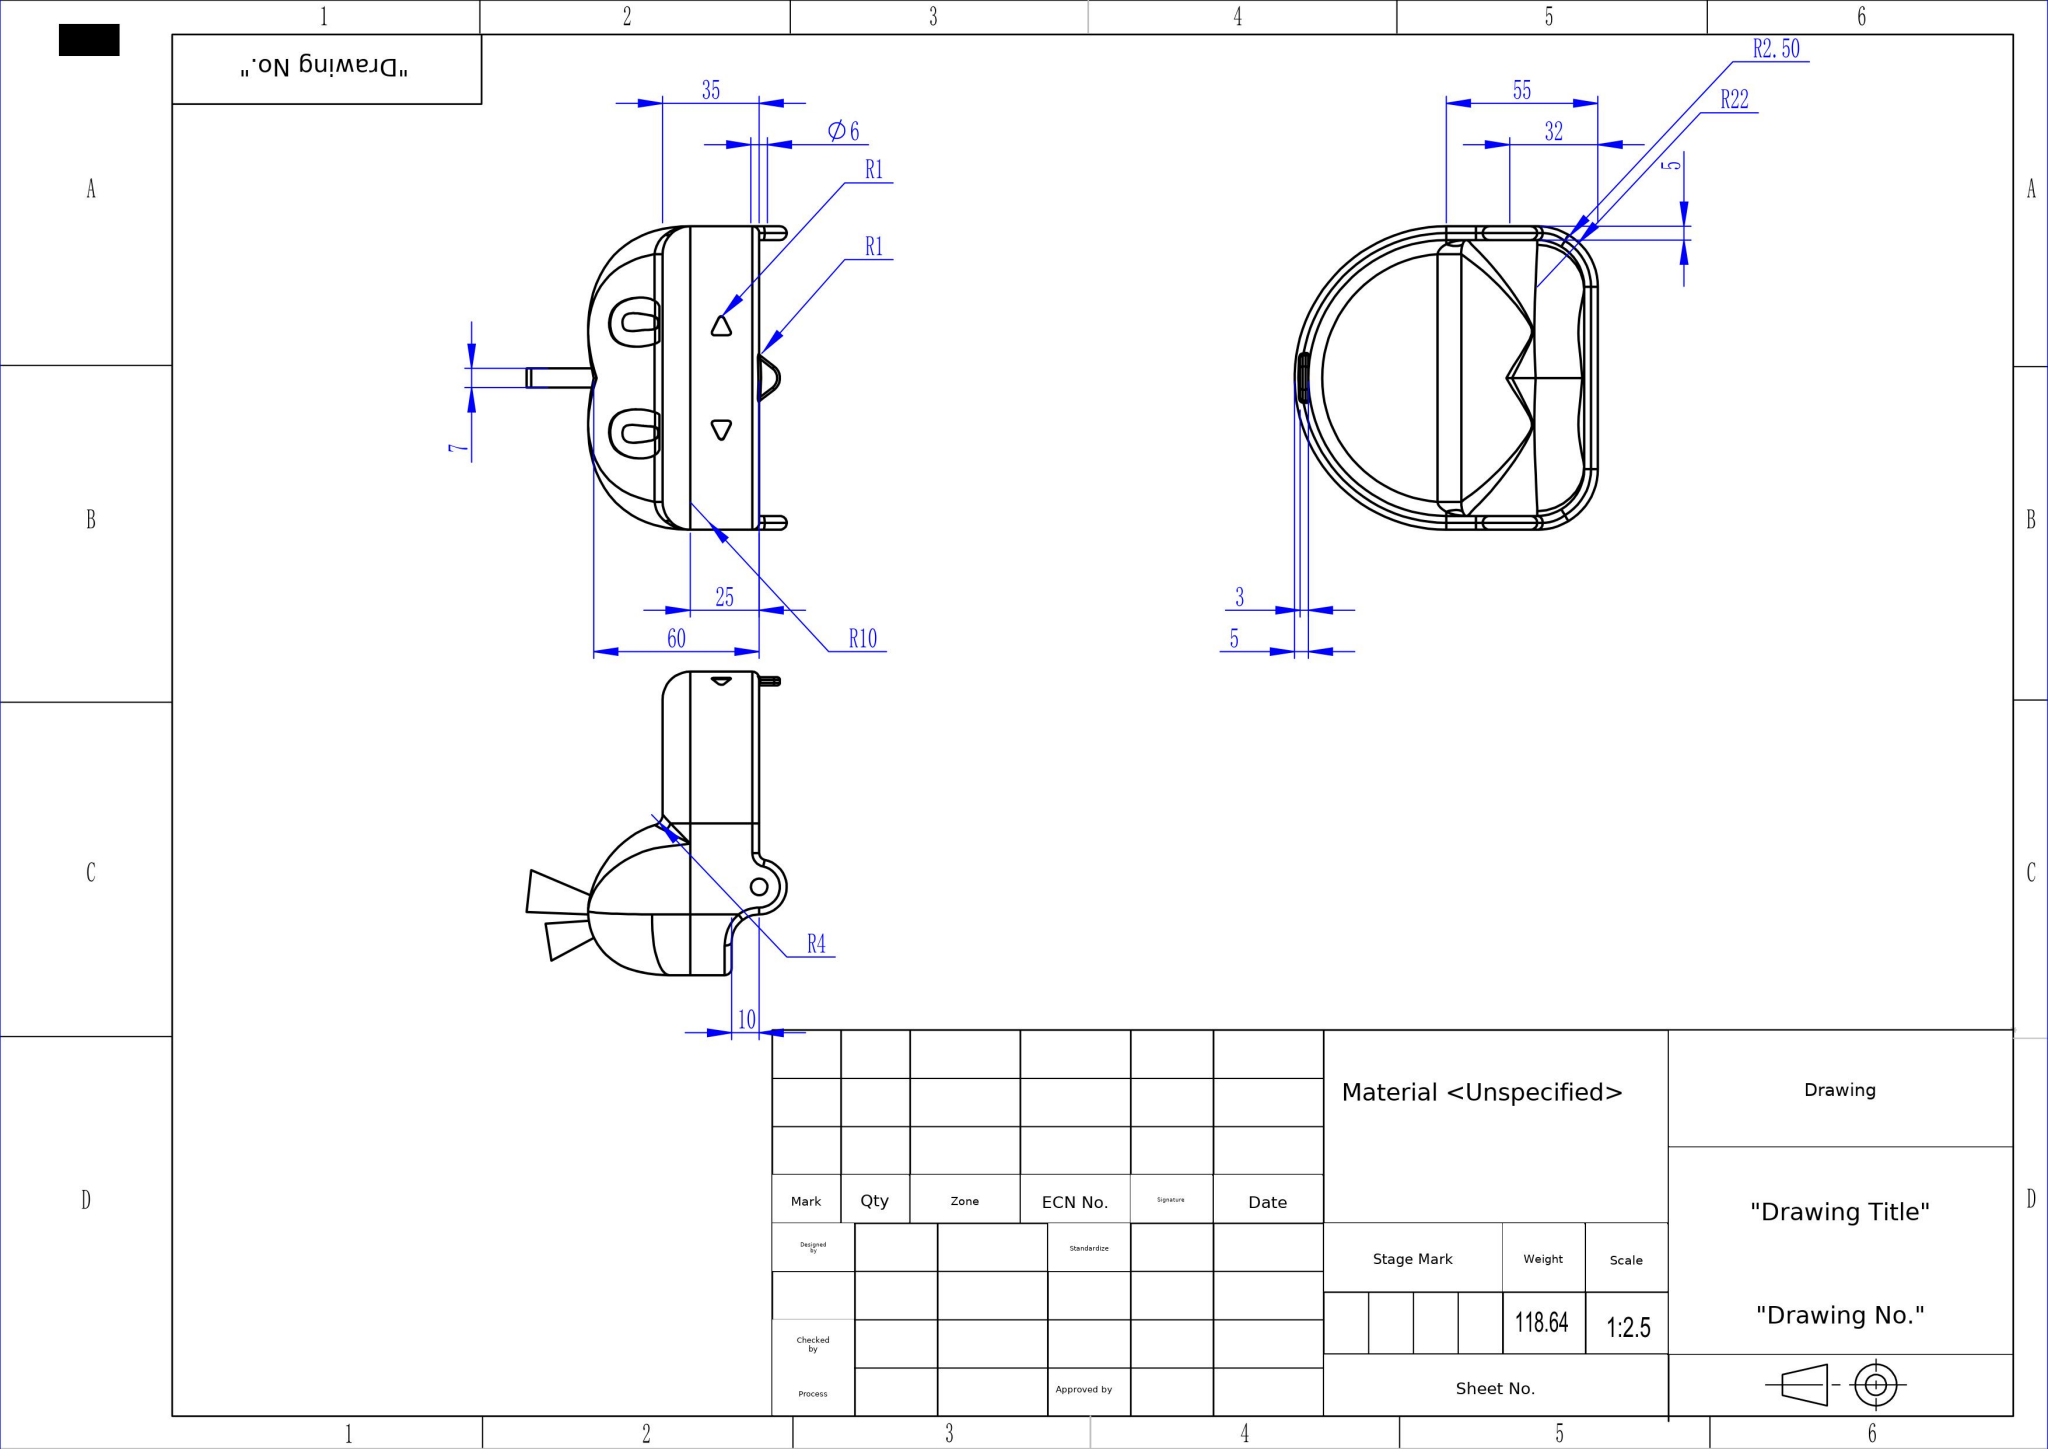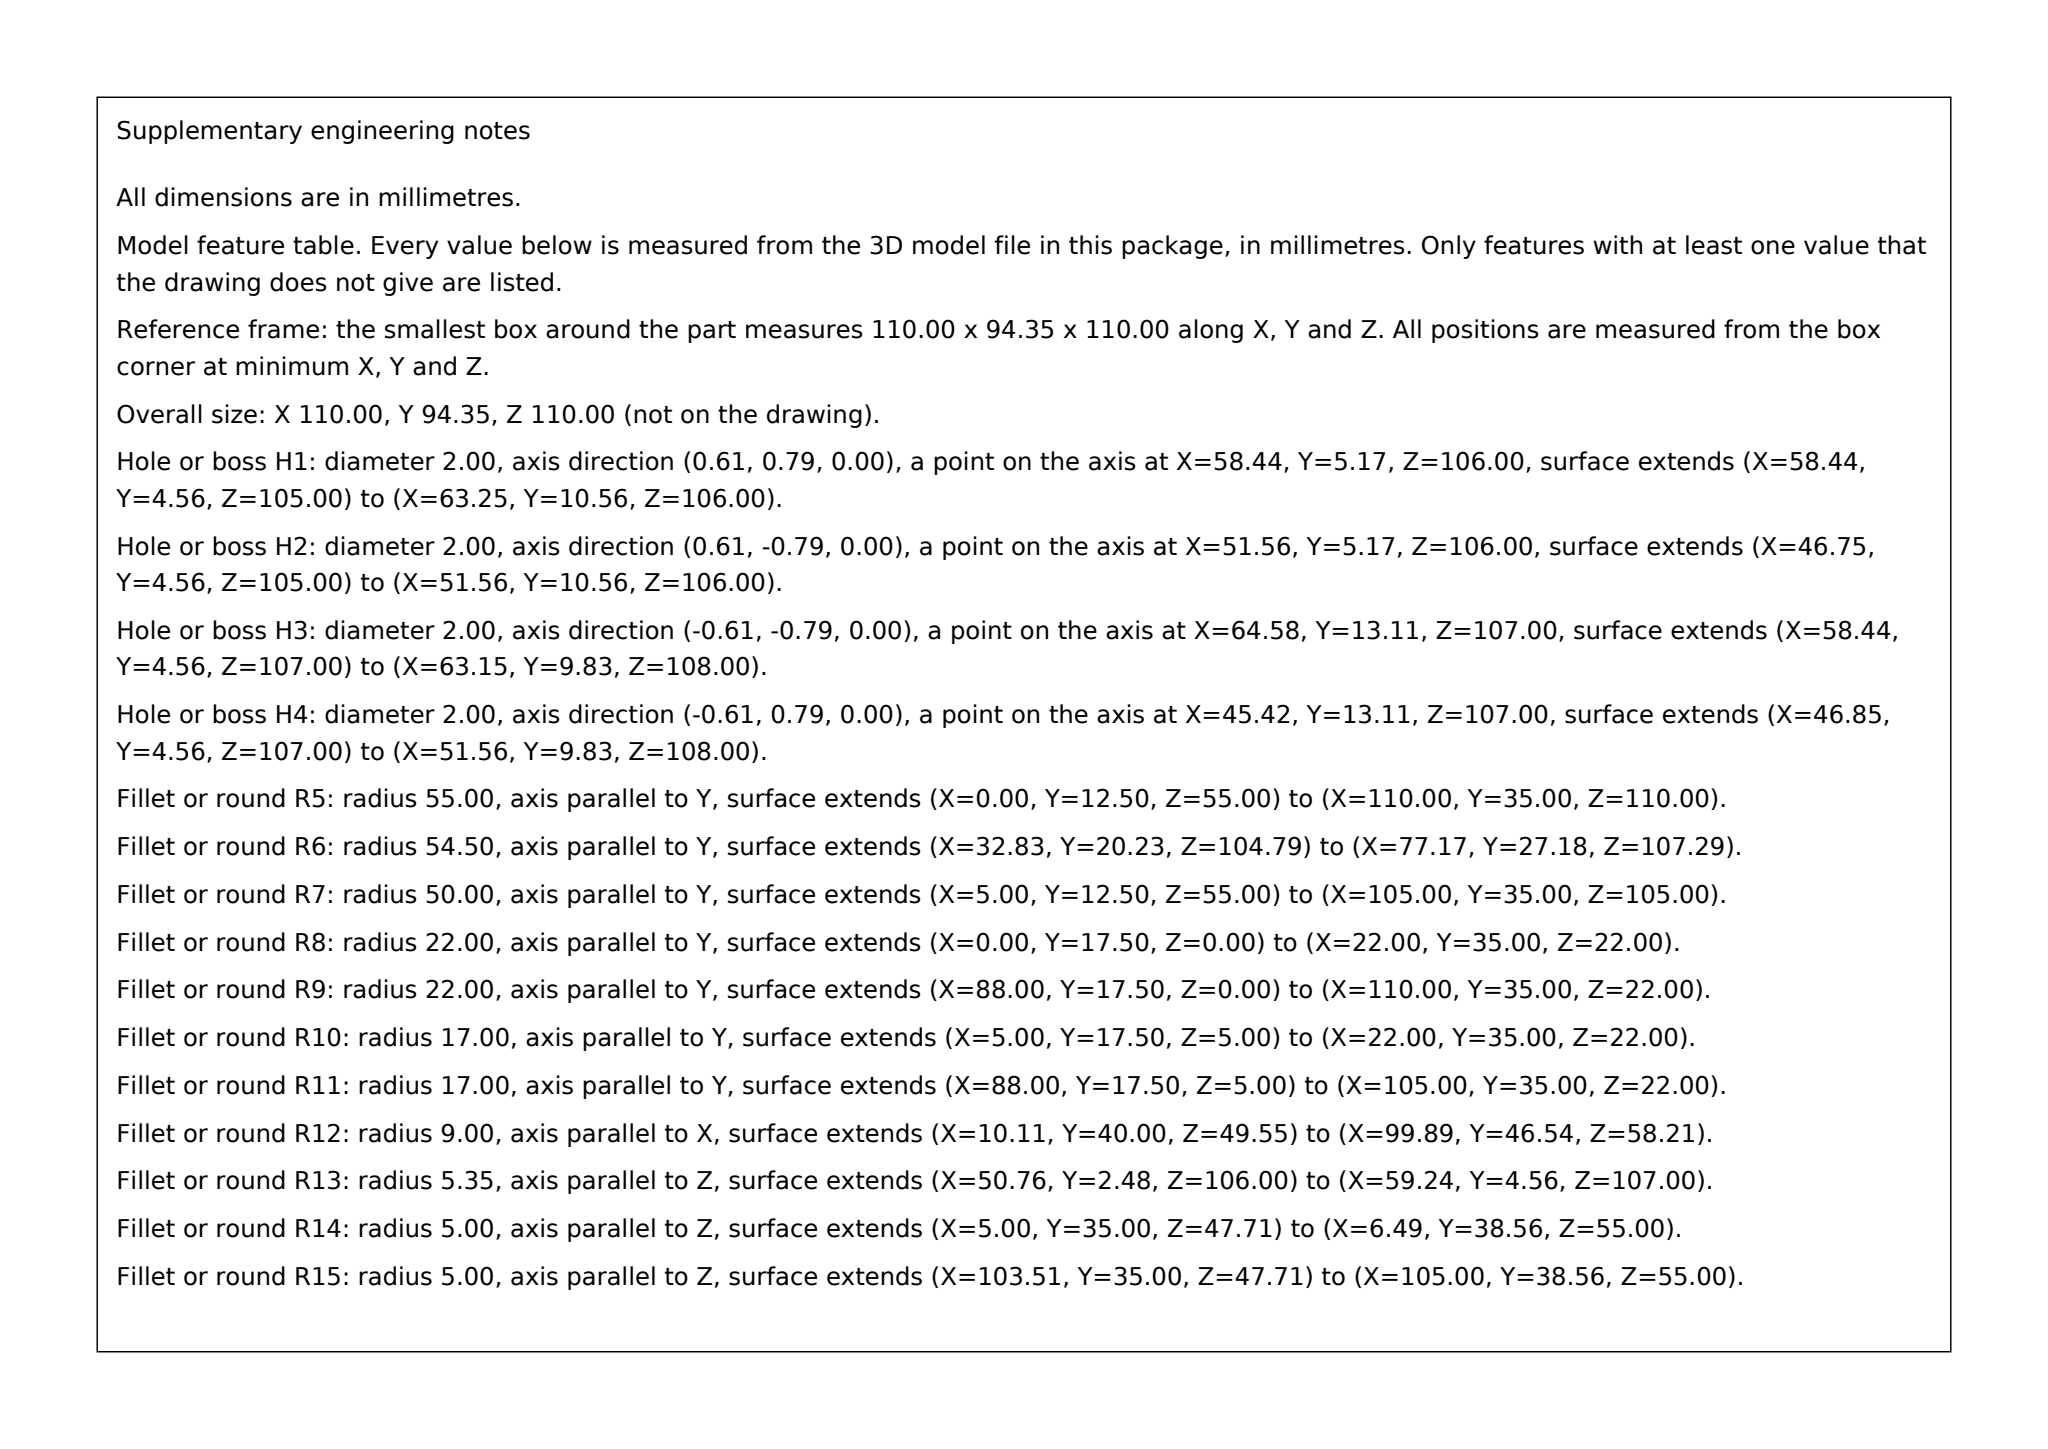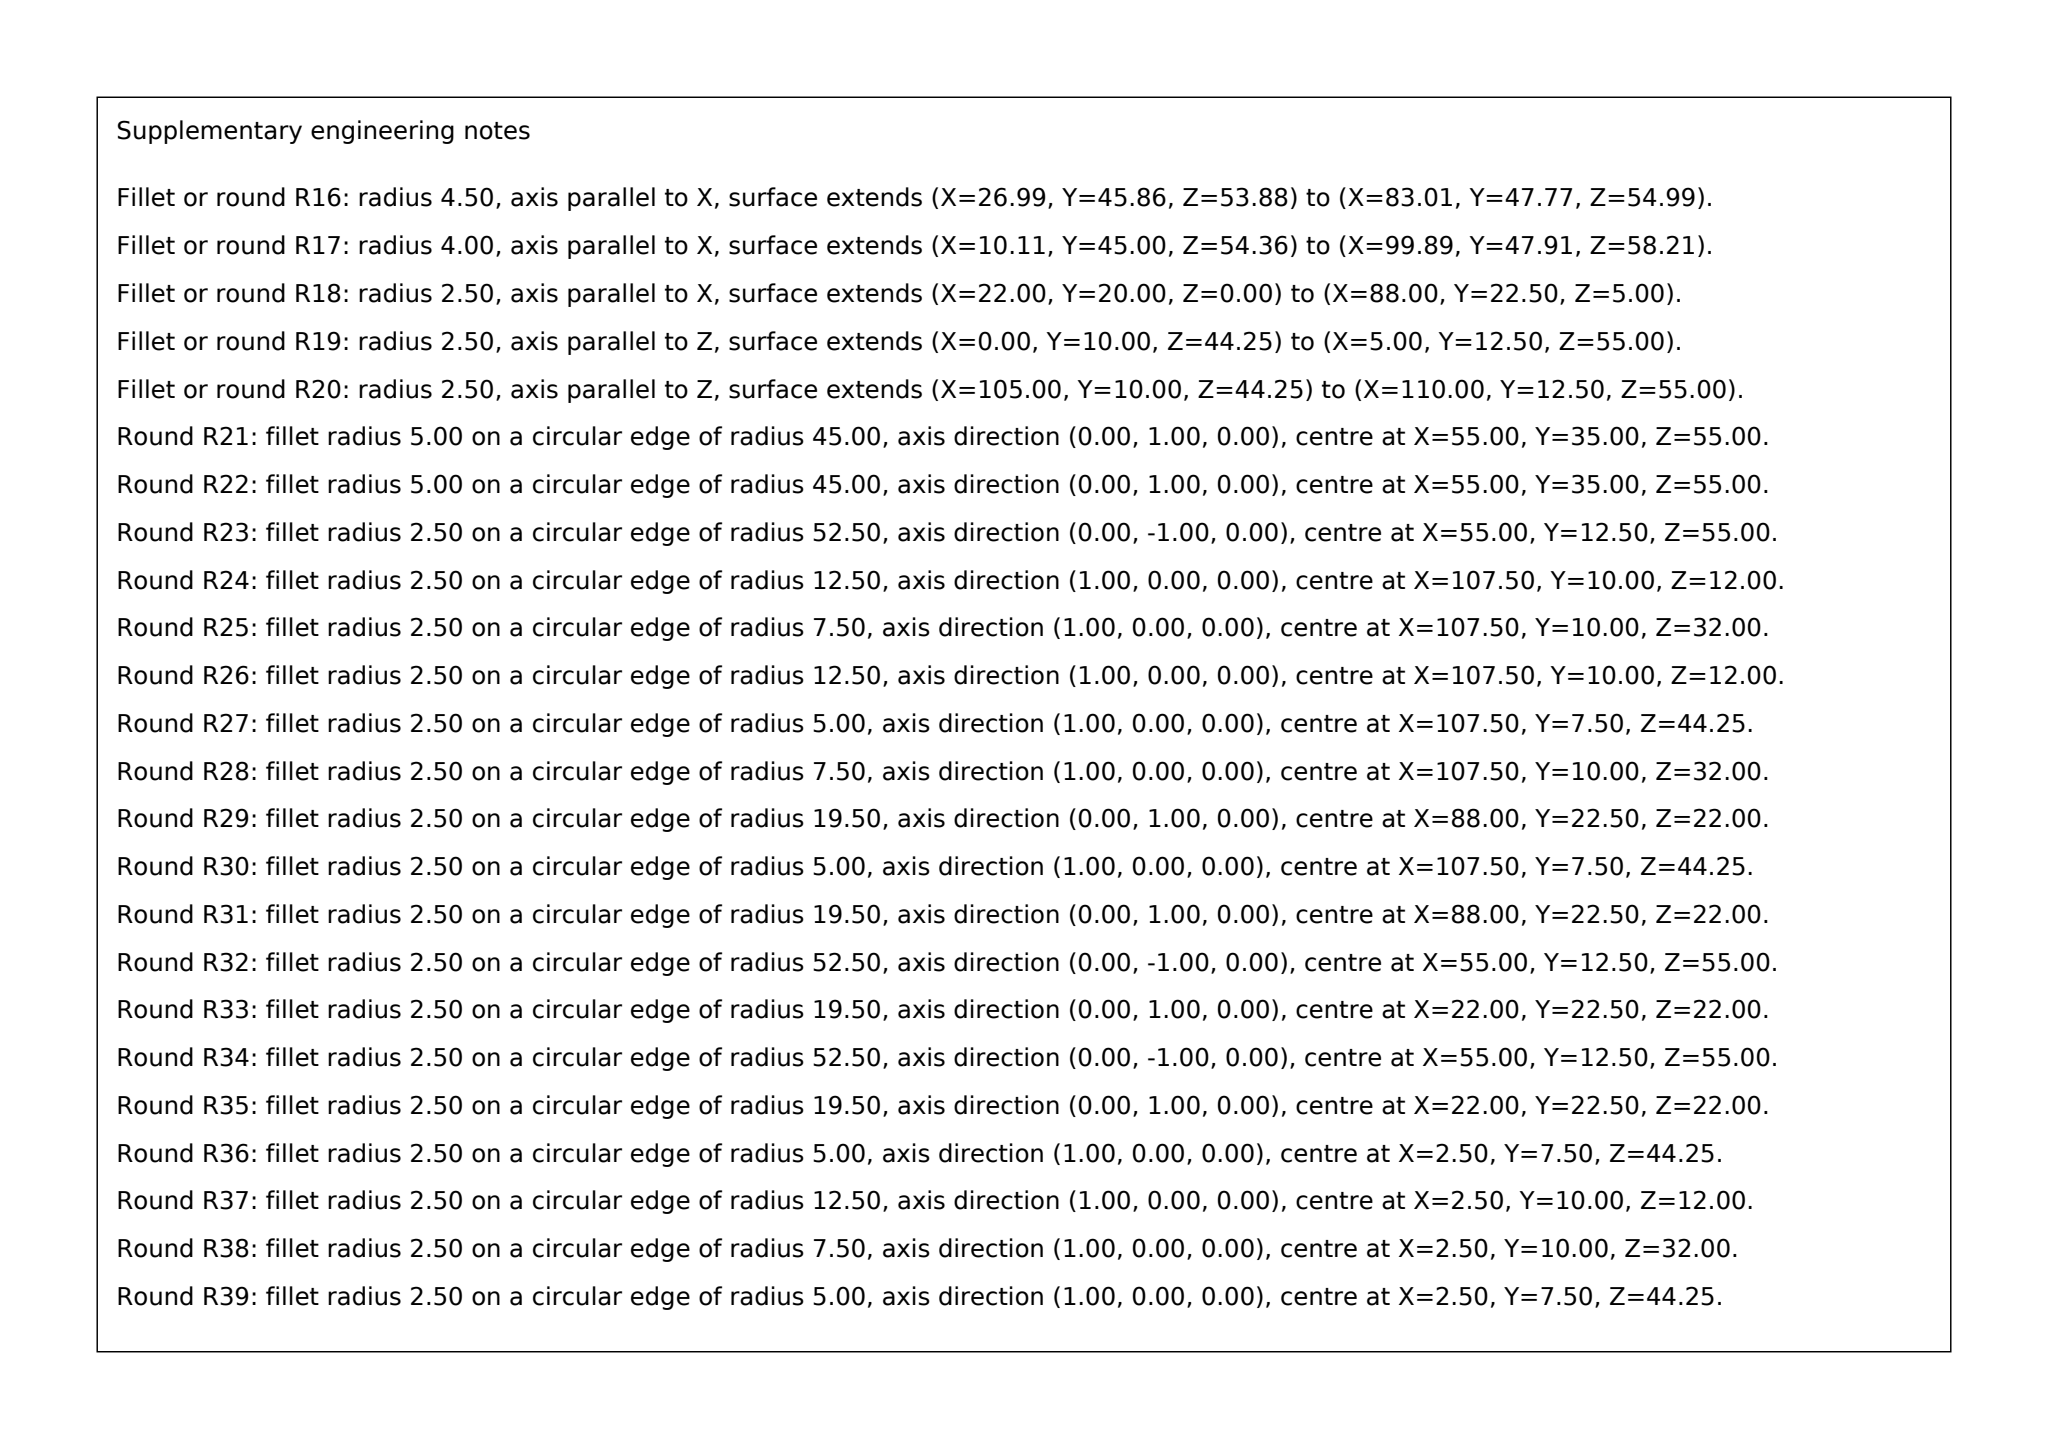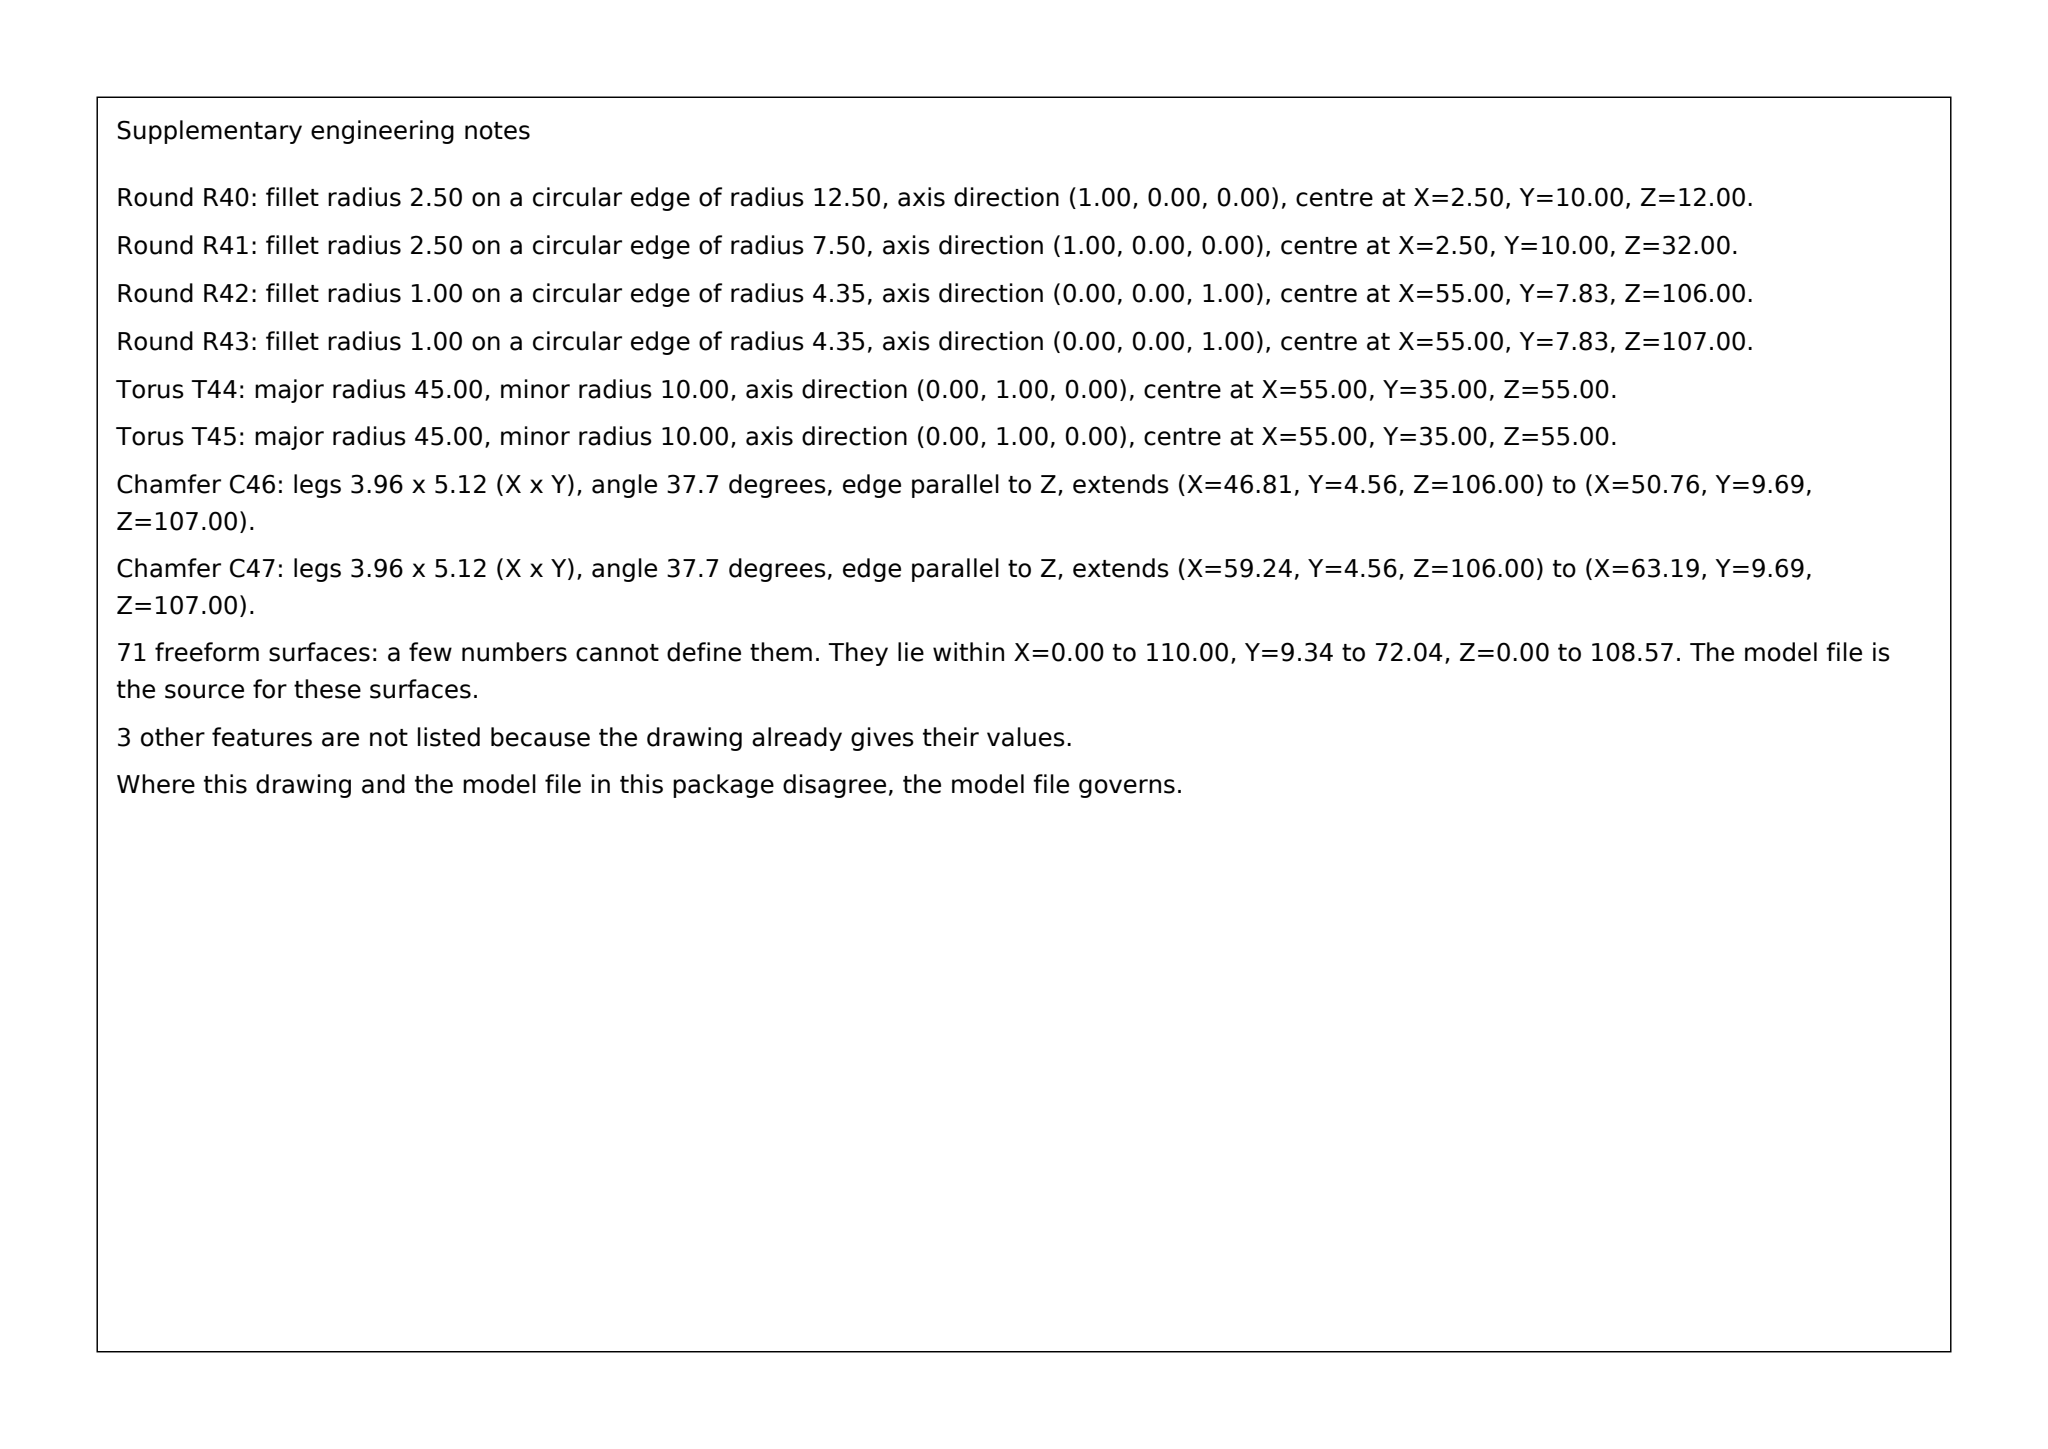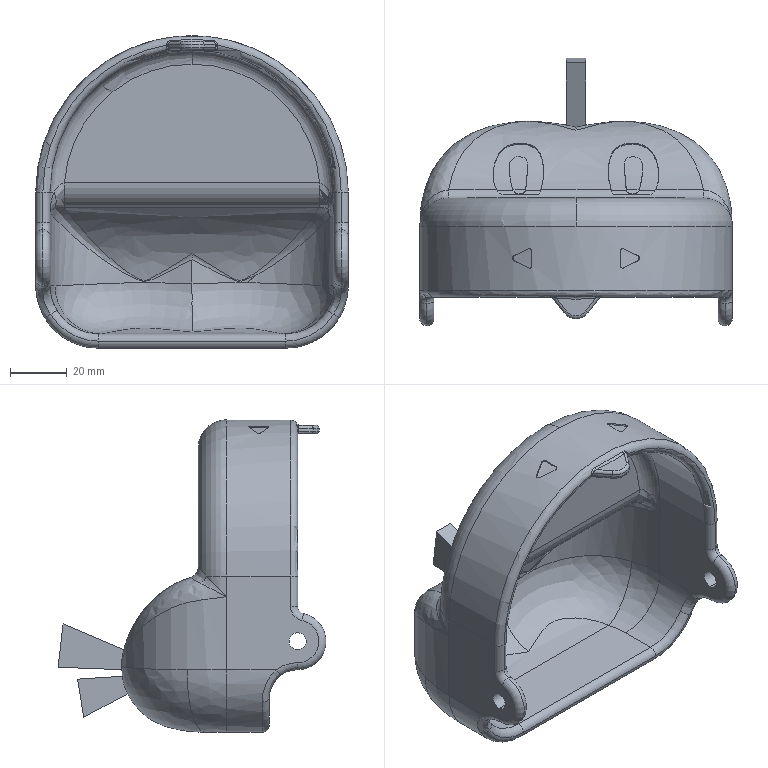Part | SolidWorks | mm | 1 solid | 152 faces | box 110 x 94.35 x 110 mm | volume 118617 mm3 | spline 71 | cylinder 33 | torus 25 | plane 23 | commonest cylinder face diameters 5 x6 6 x4 2 x4 8 x3 44 x2 20 x2 34 x2 10 x2